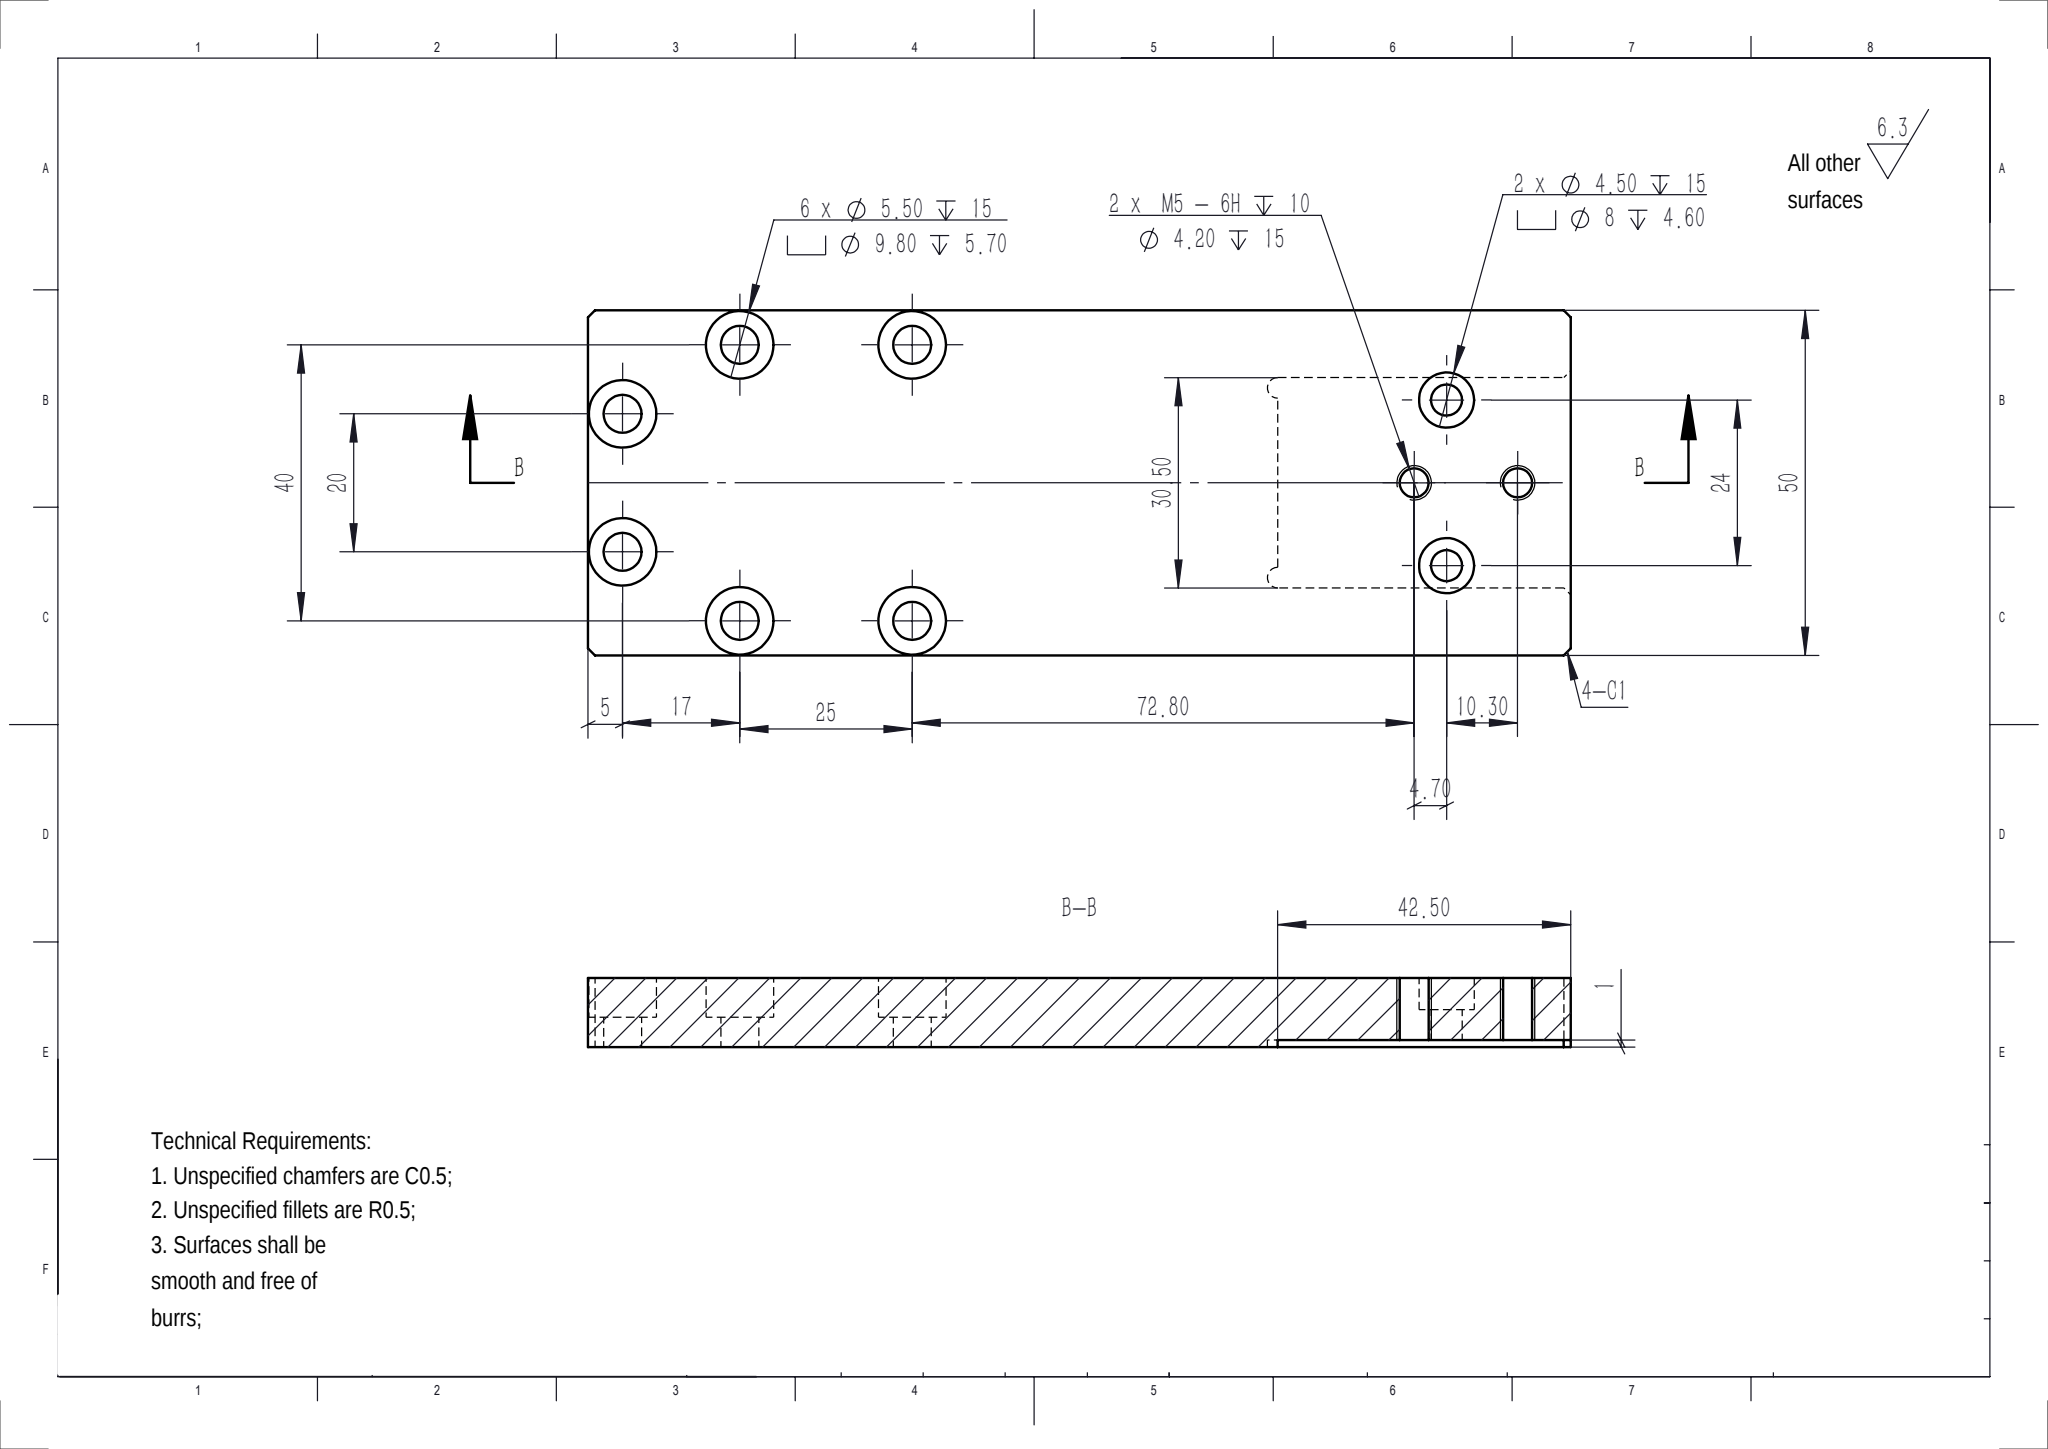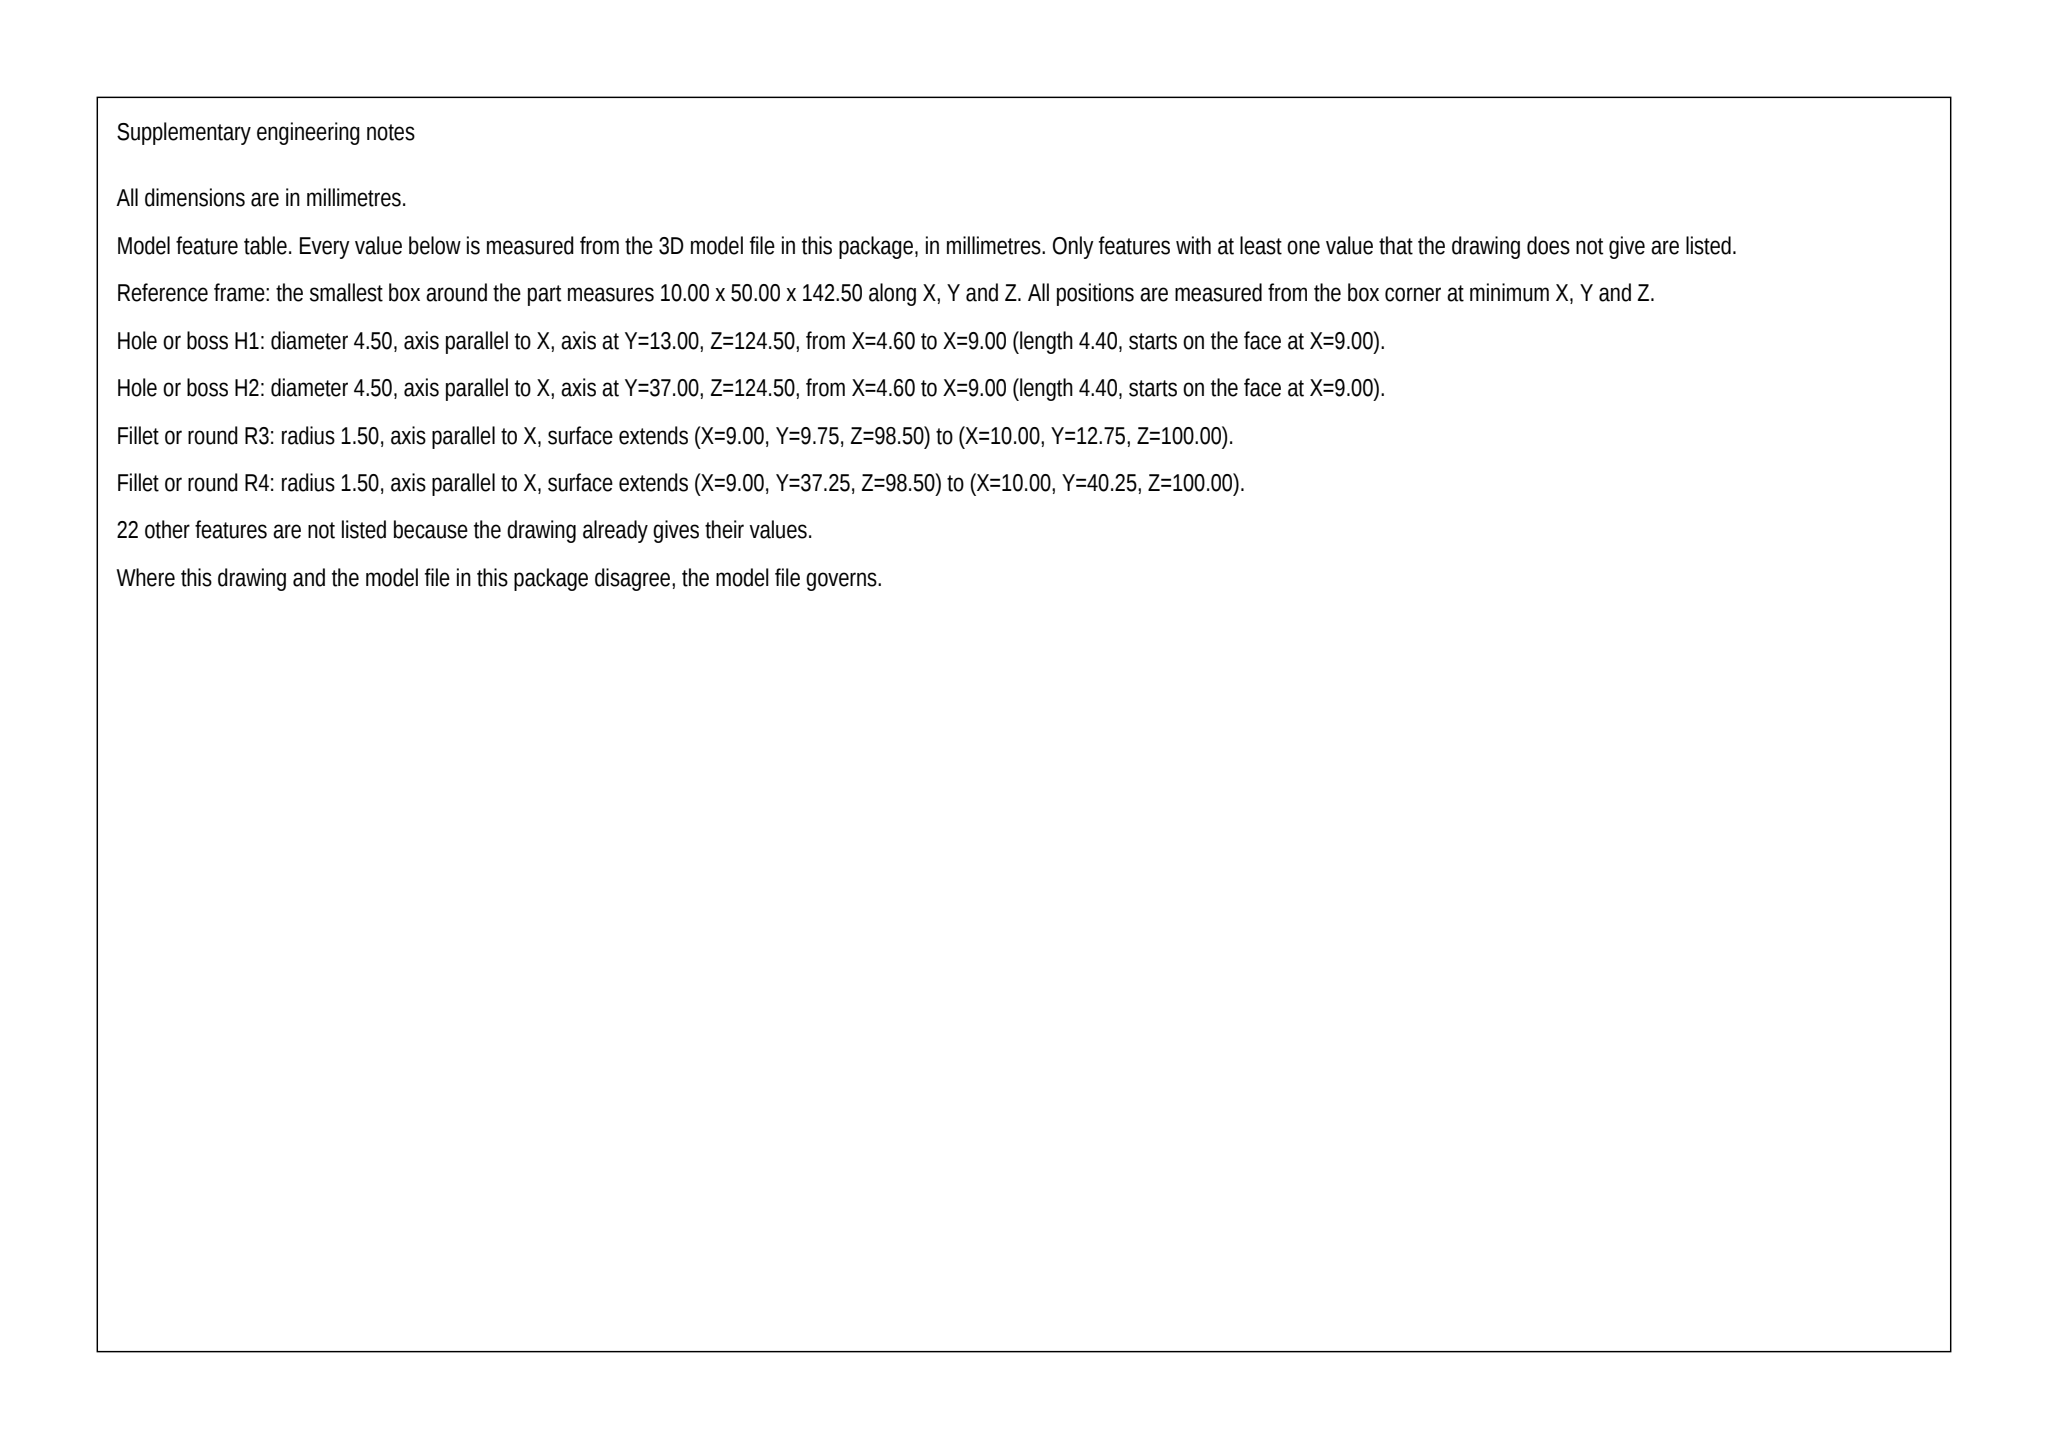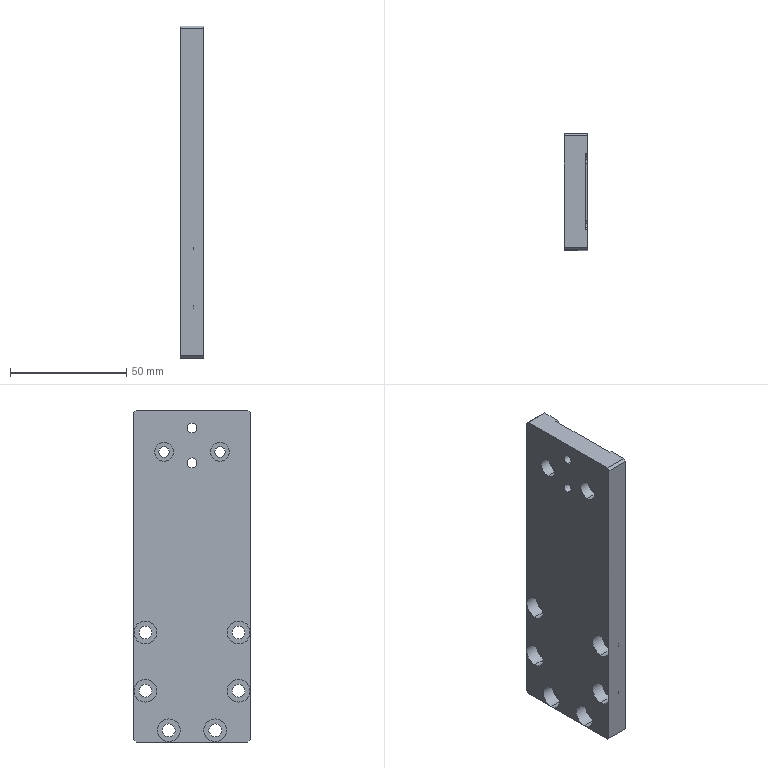Part | SolidWorks | mm | 1 solid | 64 faces | box 10 x 50 x 142.5 mm | volume 65881 mm3 | cylinder 40 | plane 24 | commonest cylinder face diameters 9.8 x12 5.5 x12 3 x4 4.2 x4 8 x4 4.5 x4
build123d program:
from build123d import *

# Parameters (mm, degrees)
SKETCH1_W                                         = 142.5
SKETCH1_H                                         = 50
BOSS_EXTRUDE1_DEPTH                               = 10
HOLE_SIZE_ACCORDING_TO_TYPE_OF_HEXAGO_D           = 5.5
HOLE_SIZE_ACCORDING_TO_TYPE_OF_HEXAGO_DEPTH       = 15
HOLE_SIZE_ACCORDING_TO_TYPE_OF_HEXAGO_CBORE_D     = 9.8
HOLE_SIZE_ACCORDING_TO_TYPE_OF_HEXAGO_CBORE_DEPTH = 5.7
HOLE_SIZE_ACCORDING_TO_TYPE_OF_HEXAGO_TIP         = 1.652
SKETCH5_W                                         = 42.5
SKETCH5_H                                         = 30.5
CUT_EXTRUDE2_DEPTH                                = 1
HOLE_SIZE_ACCORDING_TO_TYPE_OF_HE_2_D             = 4.5
HOLE_SIZE_ACCORDING_TO_TYPE_OF_HE_2_DEPTH         = 15
HOLE_SIZE_ACCORDING_TO_TYPE_OF_HE_2_CBORE_D       = 8
HOLE_SIZE_ACCORDING_TO_TYPE_OF_HE_2_CBORE_DEPTH   = 4.6
HOLE_SIZE_ACCORDING_TO_TYPE_OF_HE_2_TIP           = 1.352
M5_TAPPED_HOLE1_D                                 = 4.2
M5_TAPPED_HOLE1_DEPTH                             = 15
M5_TAPPED_HOLE1_TIP                               = 1.262
CHAMFER1_SIZE                                     = 1
SKETCH10_R                                        = 1.5
CUT_EXTRUDE3_DEPTH                                = 1


with BuildPart() as part:
    # Sketch1 → Boss-Extrude1 (new body)
    with BuildSketch(Plane(origin=(0, 0, 0), x_dir=(0, 0, -1), z_dir=(1, 0, 0))):
        Rectangle(SKETCH1_W, SKETCH1_H)
    extrude(amount=BOSS_EXTRUDE1_DEPTH)

    # Hole Size _ according to_ Type of Hexago
    with Locations(Plane.ZY):
        with Locations((-49.25, 20), (-24.25, 20), (-24.25, -20), (-49.25, -20), (-66.25, 10), (-66.25, -10)):
            CounterBoreHole(HOLE_SIZE_ACCORDING_TO_TYPE_OF_HEXAGO_D / 2, HOLE_SIZE_ACCORDING_TO_TYPE_OF_HEXAGO_CBORE_D / 2, HOLE_SIZE_ACCORDING_TO_TYPE_OF_HEXAGO_CBORE_DEPTH, depth=HOLE_SIZE_ACCORDING_TO_TYPE_OF_HEXAGO_DEPTH)
            with Locations((0, 0, -(HOLE_SIZE_ACCORDING_TO_TYPE_OF_HEXAGO_DEPTH + HOLE_SIZE_ACCORDING_TO_TYPE_OF_HEXAGO_TIP / 2))):  # 118° drill point
                Cone(0, HOLE_SIZE_ACCORDING_TO_TYPE_OF_HEXAGO_D / 2, HOLE_SIZE_ACCORDING_TO_TYPE_OF_HEXAGO_TIP, mode=Mode.SUBTRACT)

    # Sketch5 → Cut-Extrude2 (cut)
    with BuildSketch(Plane(origin=(10, 0, 0), x_dir=(0, 0, -1), z_dir=(1, 0, 0))):
        with Locations((-50, 0)):
            Rectangle(SKETCH5_W, SKETCH5_H)
    extrude(amount=-CUT_EXTRUDE2_DEPTH, mode=Mode.SUBTRACT)

    # Hole Size _ according to_ Type of He 2
    with Locations(Plane.ZY):
        with Locations((53.25, 12), (53.25, -12)):
            CounterBoreHole(HOLE_SIZE_ACCORDING_TO_TYPE_OF_HE_2_D / 2, HOLE_SIZE_ACCORDING_TO_TYPE_OF_HE_2_CBORE_D / 2, HOLE_SIZE_ACCORDING_TO_TYPE_OF_HE_2_CBORE_DEPTH, depth=HOLE_SIZE_ACCORDING_TO_TYPE_OF_HE_2_DEPTH)
            with Locations((0, 0, -(HOLE_SIZE_ACCORDING_TO_TYPE_OF_HE_2_DEPTH + HOLE_SIZE_ACCORDING_TO_TYPE_OF_HE_2_TIP / 2))):  # 118° drill point
                Cone(0, HOLE_SIZE_ACCORDING_TO_TYPE_OF_HE_2_D / 2, HOLE_SIZE_ACCORDING_TO_TYPE_OF_HE_2_TIP, mode=Mode.SUBTRACT)

    # M5 Tapped Hole1
    with Locations(Plane.ZY):
        with Locations((63.55, 0), (48.55, 0)):
            Hole(M5_TAPPED_HOLE1_D / 2, depth=M5_TAPPED_HOLE1_DEPTH)
            with Locations((0, 0, -(M5_TAPPED_HOLE1_DEPTH + M5_TAPPED_HOLE1_TIP / 2))):  # 118° drill point
                Cone(0, M5_TAPPED_HOLE1_D / 2, M5_TAPPED_HOLE1_TIP, mode=Mode.SUBTRACT)

    # Chamfer1
    chamfer1_edges = [part.edges().sort_by_distance(p)[0] for p in [
        (9.5, -15.25, 71.25),
        (9.5, 15.25, 71.25),
        (5, -25, -71.25),
        (5, -25, 71.25),
        (5, 25, 71.25),
        (5, 25, -71.25),
    ]]
    chamfer(chamfer1_edges, length=CHAMFER1_SIZE)

    # Sketch10 → Cut-Extrude3 (cut)
    with BuildSketch(Plane(origin=(10, 0, 0), x_dir=(0, 0, -1), z_dir=(1, 0, 0))):
        with Locations((-28.75, -13.75)):
            Circle(SKETCH10_R)
        with Locations((-28.75, 13.75)):
            Circle(SKETCH10_R)
    extrude(amount=-CUT_EXTRUDE3_DEPTH, mode=Mode.SUBTRACT)


solid = part.part